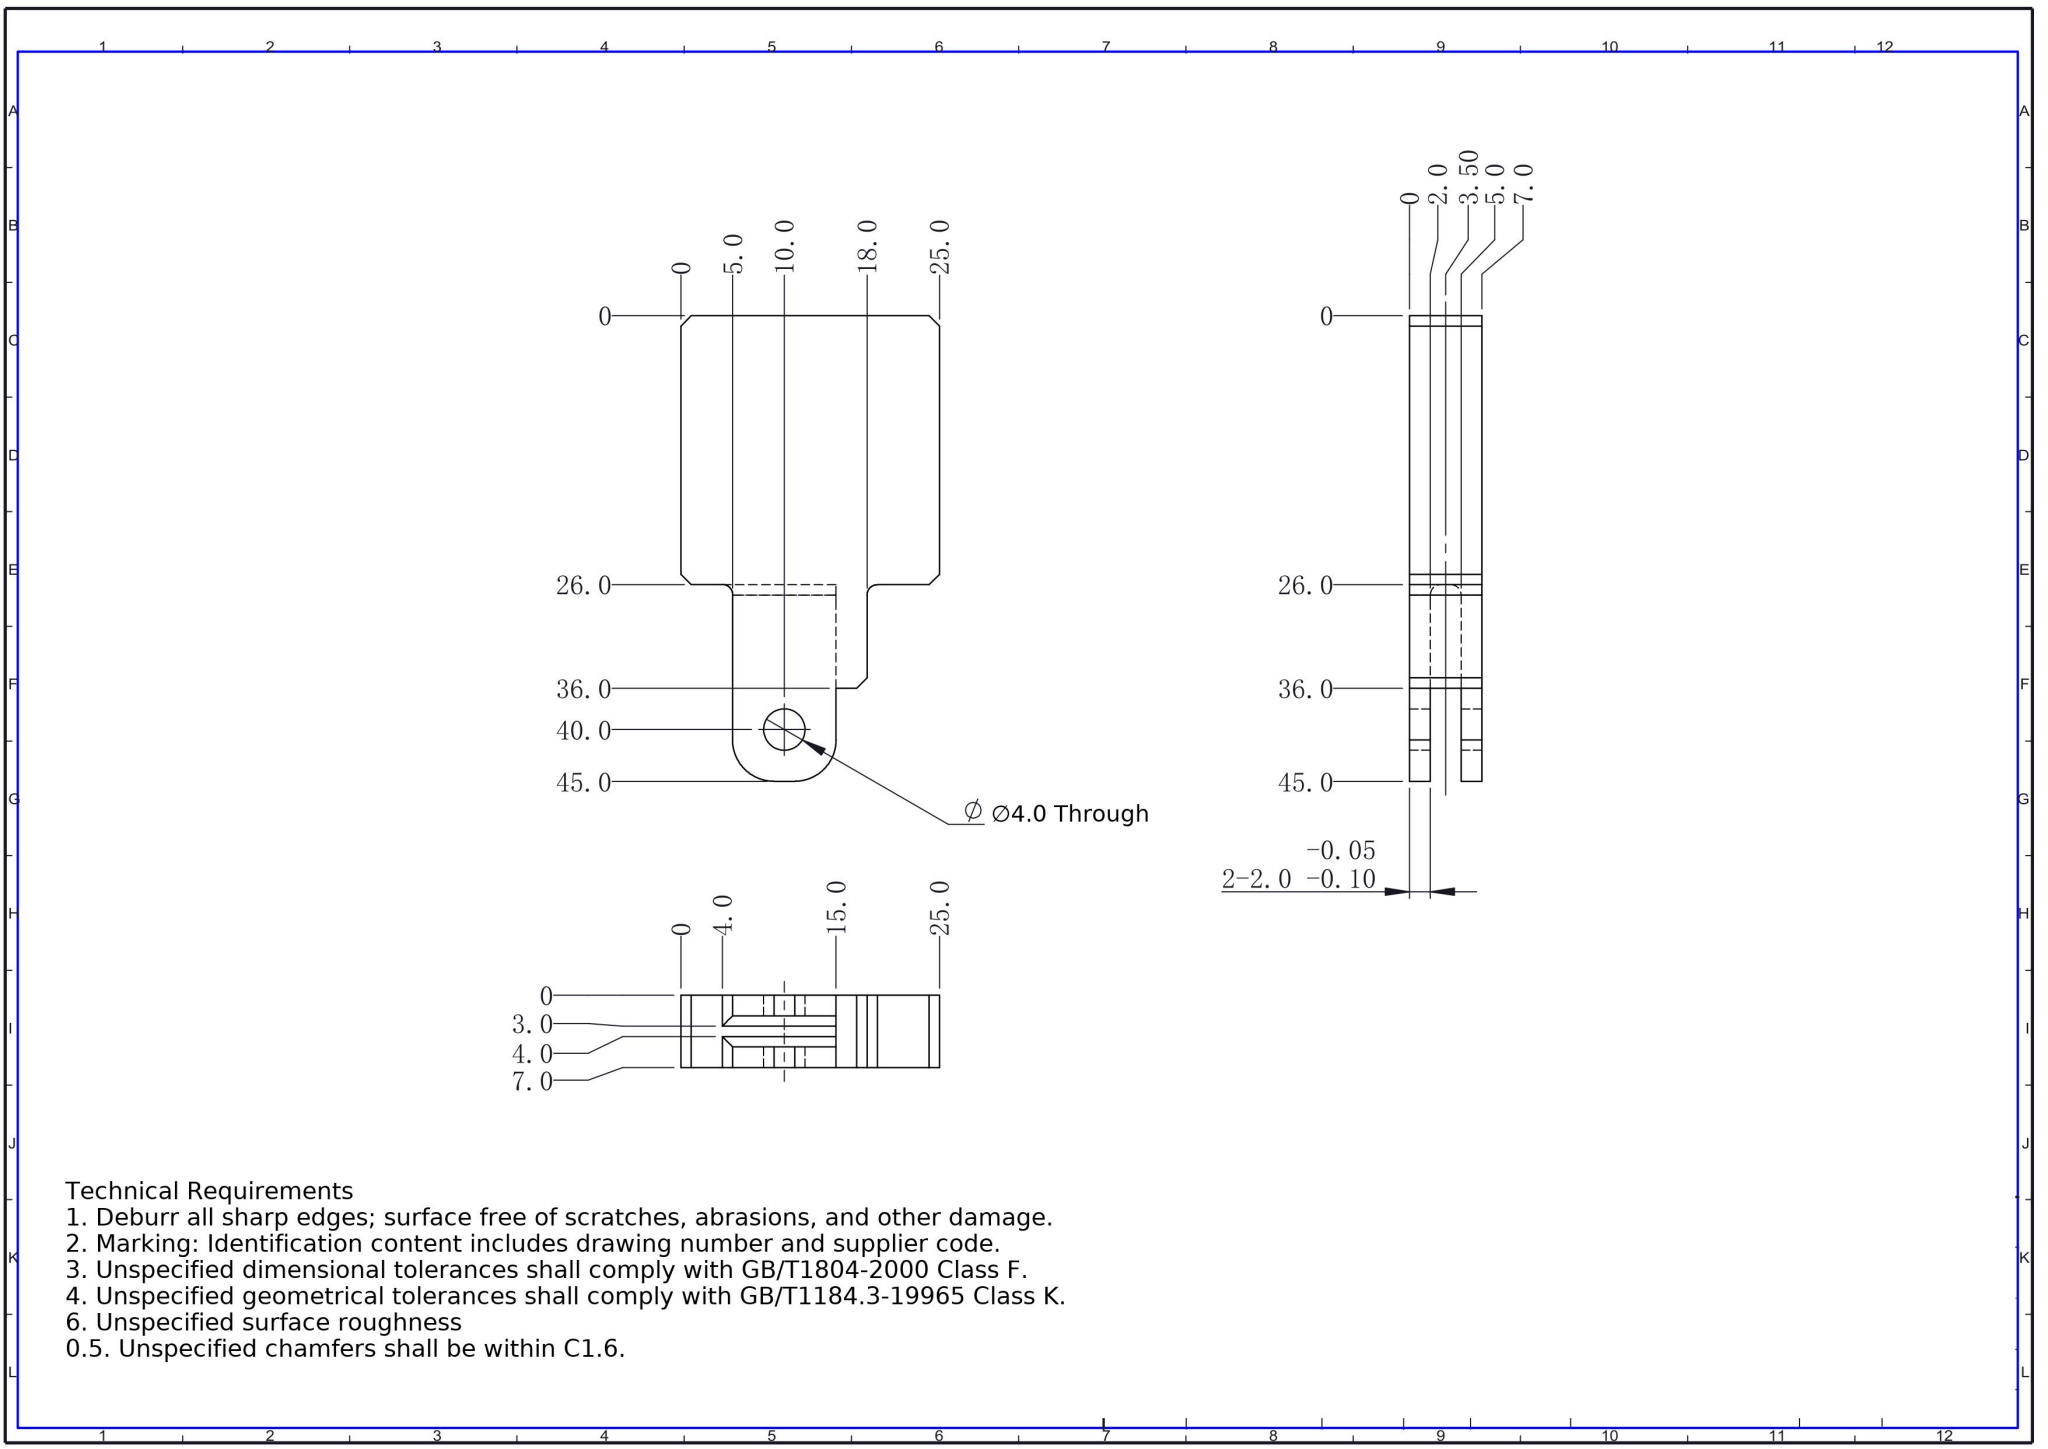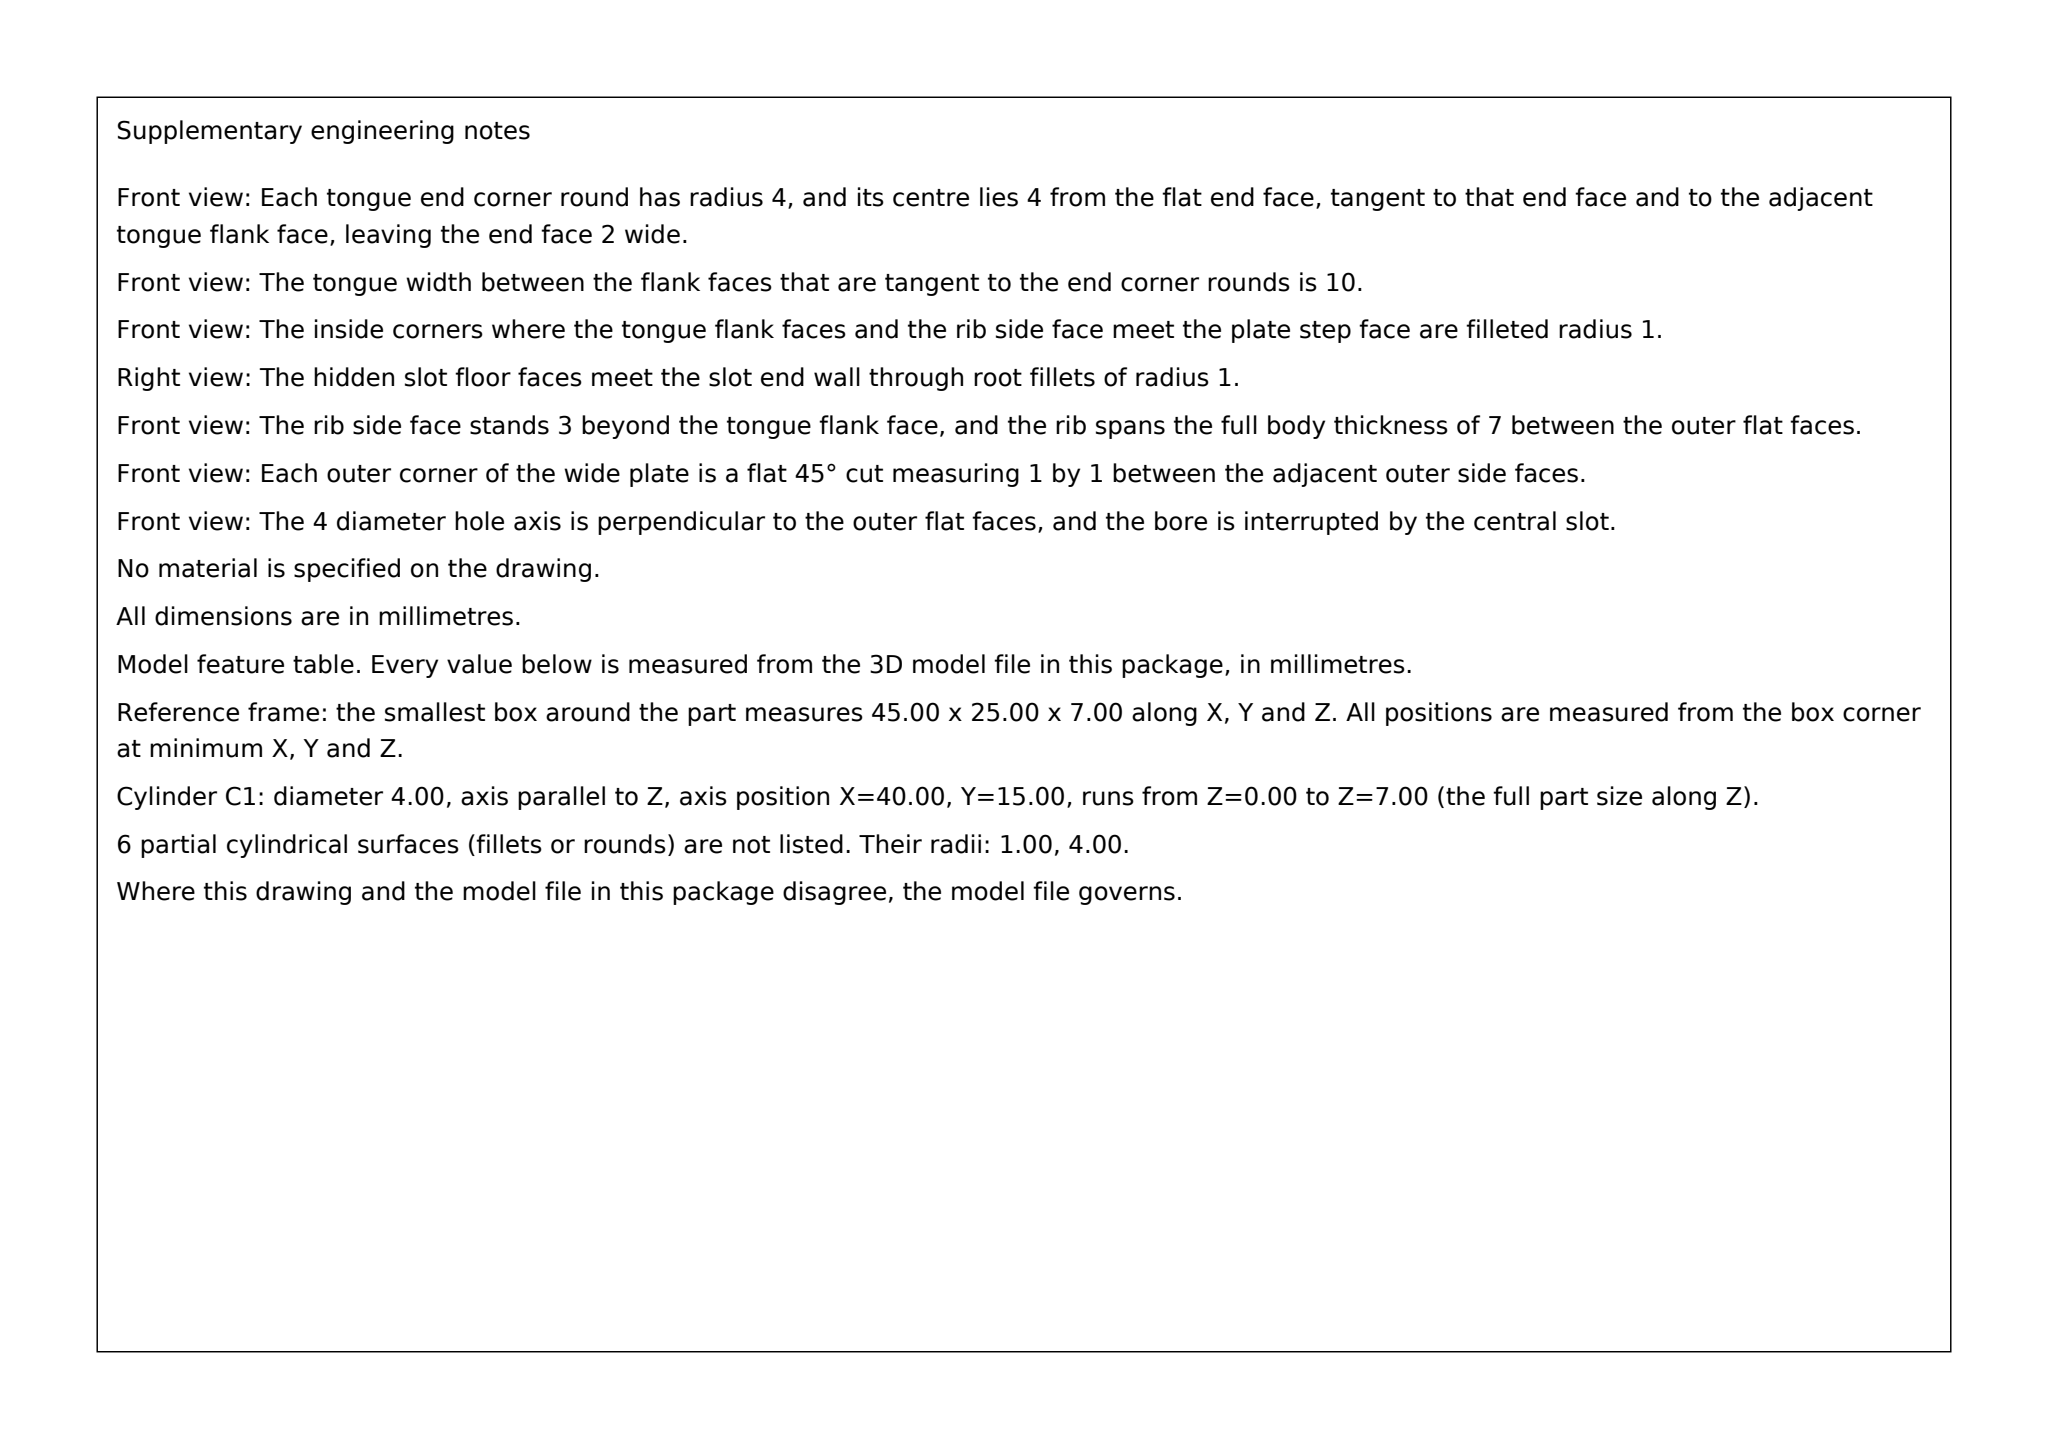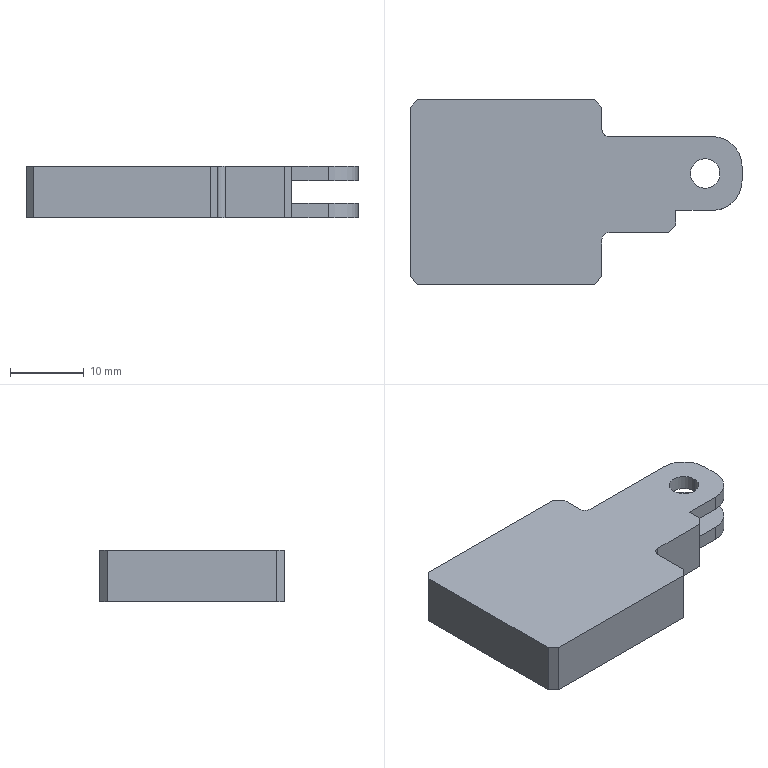Part | SolidWorks | mm | 1 solid | 36 faces | box 45 x 25 x 7 mm | volume 5432 mm3 | plane 23 | cylinder 13 | commonest cylinder face diameters 2 x5 4 x4 8 x4
Drawing notes:
0.0 END CORNERS: SHARP, NO FILLET (R0) | from the solid: No cylinders/fillet_radii near x=0; only planes x=0, y=0, y=25 meet sharp
INT SLOT BLIND END AT 26.0: 2X R1 | from the solid: Cylinders dia 2.0 axis y at (x=27.0, z=3.0) and (x=27.0, z=4.0), L=11; tangent to x=26.0 and slot walls z=2.0/5.0
26.0 SHOULDER FILLETS: 2X R1 | from the solid: Cylinders dia 2.0 axis z at (x=27.0, y=6.0) L=7 and (x=27.0, y=21.0) L=3 x2; tangent to x=26.0 and neck faces y=7.0/20.0
build123d program:
from build123d import *

# Parameters (mm, degrees)
SKETCH1_W           = 45
SKETCH1_H           = 10
BOSS_EXTRUDE1_DEPTH = 15
SKETCH2_W           = 19
SKETCH2_H           = 11.5
CUT_EXTRUDE1_DEPTH  = 15
SKETCH3_W           = 19
SKETCH3_H           = 3
CUT_EXTRUDE2_DEPTH  = 15
SKETCH4_R           = 2
CUT_EXTRUDE3_DEPTH  = 20
SKETCH5_W           = 26
SKETCH5_H           = 20
BOSS_EXTRUDE2_DEPTH = 30
SKETCH6_W           = 26
SKETCH6_H           = 11.5
CUT_EXTRUDE4_DEPTH  = 31
SKETCH7_W           = 10
SKETCH7_H           = 7
BOSS_EXTRUDE3_DEPTH = 3
MOVE_FACE1_BY       = 5
FILLET1_R           = 4
CHAMFER1_SIZE       = 1
FILLET4_R           = 1
FILLET5_R           = 1


with BuildPart() as part:
    # Sketch1 → Boss-Extrude1 (new, symmetric)
    with BuildSketch(Plane.XY):
        Rectangle(SKETCH1_W, SKETCH1_H)
    extrude(amount=BOSS_EXTRUDE1_DEPTH, both=True)

    # Sketch2 → Cut-Extrude1 (cut)
    with BuildSketch(Plane(origin=(0, 5, 0), x_dir=(1, 0, 0), z_dir=(0, 1, 0))):
        with Locations((13, 9.25)):
            Rectangle(SKETCH2_W, SKETCH2_H)
        with Locations((13, -9.25)):
            Rectangle(SKETCH2_W, SKETCH2_H)
    extrude(amount=-CUT_EXTRUDE1_DEPTH, mode=Mode.SUBTRACT)

    # Sketch3 → Cut-Extrude2 (cut)
    with BuildSketch(Plane(origin=(0, 5, 0), x_dir=(1, 0, 0), z_dir=(0, 1, 0))):
        with Locations((13, 0)):
            Rectangle(SKETCH3_W, SKETCH3_H)
    extrude(amount=-CUT_EXTRUDE2_DEPTH, mode=Mode.SUBTRACT)

    # Sketch4 → Cut-Extrude3 (cut)
    with BuildSketch(Plane(origin=(0, 0, -3.5), x_dir=(-1, 0, 0), z_dir=(0, 0, -1))):
        with Locations((-17.5, 0)):
            Circle(SKETCH4_R)
    extrude(amount=-CUT_EXTRUDE3_DEPTH, mode=Mode.SUBTRACT)

    # Sketch5 → Boss-Extrude2 (add)
    with BuildSketch(Plane.XY.offset(15)):
        with Locations((-9.5, 0)):
            Rectangle(SKETCH5_W, SKETCH5_H)
    extrude(amount=-BOSS_EXTRUDE2_DEPTH)

    # Sketch6 → Cut-Extrude4 (cut)
    with BuildSketch(Plane(origin=(0, 10, 0), x_dir=(1, 0, 0), z_dir=(0, 1, 0))):
        with Locations((-9.5, 9.25)):
            Rectangle(SKETCH6_W, SKETCH6_H)
        with Locations((-9.5, -9.25)):
            Rectangle(SKETCH6_W, SKETCH6_H)
    extrude(amount=-CUT_EXTRUDE4_DEPTH, mode=Mode.SUBTRACT)

    # Sketch7 → Boss-Extrude3 (add)
    with BuildSketch(Plane.XZ.offset(5)):
        with Locations((8.5, 0)):
            Rectangle(SKETCH7_W, SKETCH7_H)
    extrude(amount=BOSS_EXTRUDE3_DEPTH)

    # Move Face1: a face moved outward by 5.0
    extrude(part.faces().sort_by_distance((-9.5, -10, 0))[0], amount=MOVE_FACE1_BY, dir=(0, -1, 0))

    # Fillet1
    fillet1_edges = [part.edges().sort_by_distance(p)[0] for p in [
        (22.5, 5, 2.5),
        (22.5, -5, 2.5),
        (22.5, 5, -2.5),
        (22.5, -5, -2.5),
    ]]
    fillet(fillet1_edges, radius=FILLET1_R)

    # Chamfer1
    chamfer1_edges = [part.edges().sort_by_distance(p)[0] for p in [
        (3.5, -15, 0),
        (-22.5, -15, 0),
        (-22.5, 10, 0),
        (3.5, 10, 0),
        (13.5, -8, 0),
    ]]
    chamfer(chamfer1_edges, length=CHAMFER1_SIZE)

    # Fillet4
    fillet4_edges = [part.edges().sort_by_distance(p)[0] for p in [
        (3.5, 0, 1.5),
        (3.5, 0, -1.5),
    ]]
    fillet(fillet4_edges, radius=FILLET4_R)

    # Fillet5
    fillet5_edges = [part.edges().sort_by_distance(p)[0] for p in [
        (3.5, 5, -2),
        (3.5, 5, 2),
        (3.5, -8, 0),
    ]]
    fillet(fillet5_edges, radius=FILLET5_R)


solid = part.part